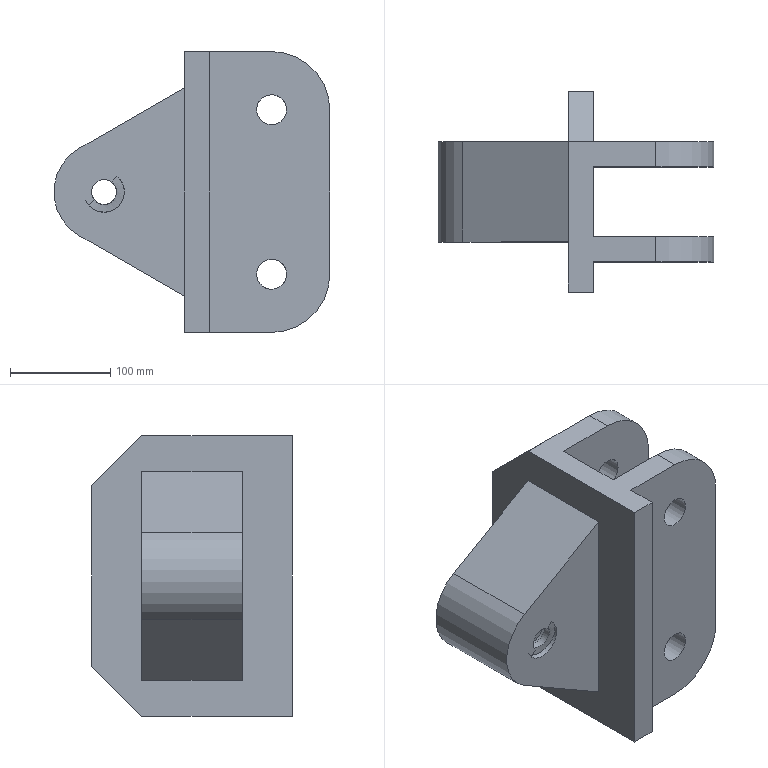Component | NX | MOVING_BLOCK | 1 solid | 33 faces | volume 4482392 mm3 | plane 20 | cylinder 10 | spline 3 | commonest cylinder face diameters 116 x4 30 x4 25 x1 100 x1